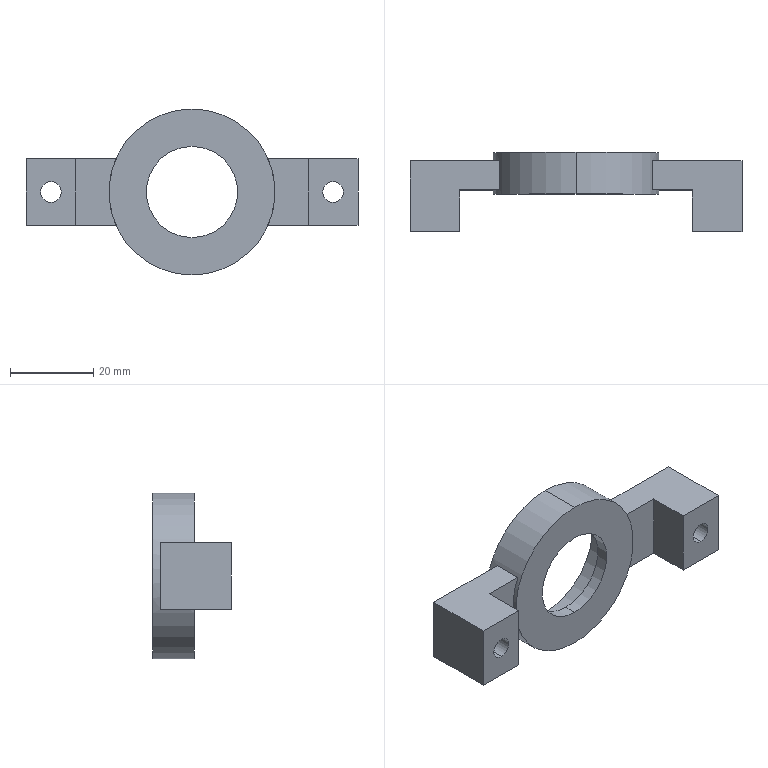Component | SolidWorks | BearingHousing-2 | 1 solid | 33 faces | box 80 x 19 x 40 mm | volume 12982 mm3 | plane 19 | cylinder 14 | commonest cylinder face diameters 10 x4 5 x4 32 x2 40 x2 22 x2 | material A-Glass Fiber
build123d program:
from build123d import *

# Parameters (mm, degrees)
BOSS_EXTRUDE1_DEPTH      = 7
BOSS_EXTRUDE1_DEPTH_BACK = 3
SKETCH1_R                = 20
SKETCH1_R_2              = 11
BOSS_EXTRUDE2_START      = -2
BOSS_EXTRUDE2_DEPTH      = 7
SKETCH3_W                = 12
SKETCH3_H                = 16
BOSS_EXTRUDE3_DEPTH      = 12
SKETCH4_R                = 2.5
CUT_EXTRUDE1_DEPTH       = 49.59
SKETCH5_R                = 5
CUT_EXTRUDE2_DEPTH       = 5
SKETCH6_R                = 16
CUT_EXTRUDE3_DEPTH       = 7


with BuildPart() as part:
    # Sketch1 → Boss-Extrude1 (new, two sides: drawn at the far end of the back side and taken through both)
    with BuildSketch(Plane(origin=(0, 0, 0), x_dir=(1, 0, 0), z_dir=(0, 1, 0)).offset(-BOSS_EXTRUDE1_DEPTH_BACK)):
        with Locations(Location((0, 0, 0), (0, 0, 270))):
            Circle(SKETCH1_R)
        with Locations(Location((0, 0, 0), (0, 0, 270))):
            Circle(SKETCH1_R_2, mode=Mode.SUBTRACT)
    extrude(amount=BOSS_EXTRUDE1_DEPTH + BOSS_EXTRUDE1_DEPTH_BACK)

    # Sketch2 → Boss-Extrude2 (add)
    with BuildSketch(Plane(origin=(0, 0, 0), x_dir=(1, 0, 0), z_dir=(0, 1, 0)).offset(BOSS_EXTRUDE2_START)):
        with BuildLine():
            Line((40, 8), (18.33, 8))
            ThreePointArc((18.33, 8), (20, 0), (18.33, -8))
            Line((18.33, -8), (40, -8))
            Line((40, -8), (40, 8))
        make_face()
    boss_extrude2 = extrude(amount=BOSS_EXTRUDE2_DEPTH)

    # Sketch3 → Boss-Extrude3 (add)
    with BuildSketch(Plane(origin=(0, 0, 0), x_dir=(1, 0, 0), z_dir=(0, 1, 0))):
        with Locations((34, 0)):
            Rectangle(SKETCH3_W, SKETCH3_H)
    boss_extrude3 = extrude(amount=-BOSS_EXTRUDE3_DEPTH)

    # Sketch4 → Cut-Extrude1 (cut, through all)
    with BuildSketch(Plane.XZ.offset(12)):
        with Locations(Location((34, 0, 0), (0, 0, 270))):
            Circle(SKETCH4_R)
    cut_extrude1 = extrude(amount=-CUT_EXTRUDE1_DEPTH, mode=Mode.SUBTRACT)

    # Sketch5 → Cut-Extrude2 (cut)
    with BuildSketch(Plane(origin=(0, 5, 0), x_dir=(1, 0, 0), z_dir=(0, 1, 0))):
        with Locations(Location((34, 0, 0), (0, 0, 270))):
            Circle(SKETCH5_R)
    cut_extrude2 = extrude(amount=-CUT_EXTRUDE2_DEPTH, mode=Mode.SUBTRACT)

    # Mirror1: Boss-Extrude2, Boss-Extrude3, Cut-Extrude1, Cut-Extrude2 across plane
    add(boss_extrude2.mirror(Plane(origin=(0, 0, 0), x_dir=(0, 0, 1), z_dir=(1, 0, 0))))
    add(boss_extrude3.mirror(Plane(origin=(0, 0, 0), x_dir=(0, 0, 1), z_dir=(1, 0, 0))))
    add(cut_extrude1.mirror(Plane(origin=(0, 0, 0), x_dir=(0, 0, 1), z_dir=(1, 0, 0))), mode=Mode.SUBTRACT)
    add(cut_extrude2.mirror(Plane(origin=(0, 0, 0), x_dir=(0, 0, 1), z_dir=(1, 0, 0))), mode=Mode.SUBTRACT)

    # Sketch6 → Cut-Extrude3 (cut)
    with BuildSketch(Plane(origin=(0, 7, 0), x_dir=(1, 0, 0), z_dir=(0, 1, 0))):
        with Locations(Location((0, 0, 0), (0, 0, 270))):
            Circle(SKETCH6_R)
    extrude(amount=-CUT_EXTRUDE3_DEPTH, mode=Mode.SUBTRACT)


solid = part.part

# Placed as in the assembly
solid = solid.moved(Location((-96.534, 130.266, -166.507), (0, 0, 0)))
STEP:
#1=COLOUR_RGB('',0.7922,0.8196,0.9333);
#2=FILL_AREA_STYLE_COLOUR('',#1);
#3=FILL_AREA_STYLE('',(#2));
#4=SURFACE_STYLE_FILL_AREA(#3);
#5=SURFACE_SIDE_STYLE('',(#4));
#6=SURFACE_STYLE_USAGE(.BOTH.,#5);
#7=PRESENTATION_STYLE_ASSIGNMENT((#6));
#8=CARTESIAN_POINT('',(-3.801,5.129,-7.185));
#9=VERTEX_POINT('',#8);
#10=CARTESIAN_POINT('',(-3.801,5.129,-5.925));
#11=VERTEX_POINT('',#10);
#12=CARTESIAN_POINT('',(-3.801,5.129,-6.555));
#13=DIRECTION('',(0.,1.,0.));
#14=DIRECTION('',(0.,0.,1.));
#15=AXIS2_PLACEMENT_3D('',#12,#13,#14);
#16=CIRCLE('',#15,0.6299);
#17=EDGE_CURVE('',#9,#11,#16,.T.);
#18=ORIENTED_EDGE('',*,*,#17,.F.);
#19=CARTESIAN_POINT('',(-3.801,5.404,-7.185));
#20=VERTEX_POINT('',#19);
#21=CARTESIAN_POINT('',(-3.801,5.129,-7.185));
#22=DIRECTION('',(0.,1.,0.));
#23=VECTOR('',#22,39.37);
#24=LINE('',#21,#23);
#25=EDGE_CURVE('',#9,#20,#24,.T.);
#26=ORIENTED_EDGE('',*,*,#25,.T.);
#27=CARTESIAN_POINT('',(-3.801,5.404,-5.925));
#28=VERTEX_POINT('',#27);
#29=CARTESIAN_POINT('',(-3.801,5.404,-6.555));
#30=DIRECTION('',(0.,1.,0.));
#31=DIRECTION('',(0.,0.,1.));
#32=AXIS2_PLACEMENT_3D('',#29,#30,#31);
#33=CIRCLE('',#32,0.6299);
#34=EDGE_CURVE('',#20,#28,#33,.T.);
#35=ORIENTED_EDGE('',*,*,#34,.T.);
#36=CARTESIAN_POINT('',(-3.801,5.129,-5.925));
#37=DIRECTION('',(0.,1.,0.));
#38=VECTOR('',#37,39.37);
#39=LINE('',#36,#38);
#40=EDGE_CURVE('',#11,#28,#39,.T.);
#41=ORIENTED_EDGE('',*,*,#40,.F.);
#42=EDGE_LOOP('',(#18,#26,#35,#41));
#43=FACE_OUTER_BOUND('',#42,.T.);
#44=CARTESIAN_POINT('',(-3.801,5.129,-6.555));
#45=DIRECTION('',(0.,1.,0.));
#46=DIRECTION('',(0.,0.,1.));
#47=AXIS2_PLACEMENT_3D('',#44,#45,#46);
#48=CYLINDRICAL_SURFACE('',#47,0.6299);
#49=ADVANCED_FACE('',(#43),#48,.F.);
#50=CARTESIAN_POINT('',(-5.139,5.129,-6.359));
#51=VERTEX_POINT('',#50);
#52=CARTESIAN_POINT('',(-5.139,5.129,-6.752));
#53=VERTEX_POINT('',#52);
#54=CARTESIAN_POINT('',(-5.139,5.129,-6.555));
#55=DIRECTION('',(0.,-1.,0.));
#56=DIRECTION('',(0.,0.,1.));
#57=AXIS2_PLACEMENT_3D('',#54,#55,#56);
#58=CIRCLE('',#57,0.1969);
#59=EDGE_CURVE('',#51,#53,#58,.T.);
#60=ORIENTED_EDGE('',*,*,#59,.T.);
#61=CARTESIAN_POINT('',(-5.139,5.325,-6.752));
#62=VERTEX_POINT('',#61);
#63=CARTESIAN_POINT('',(-5.139,5.129,-6.752));
#64=DIRECTION('',(0.,1.,0.));
#65=VECTOR('',#64,39.37);
#66=LINE('',#63,#65);
#67=EDGE_CURVE('',#53,#62,#66,.T.);
#68=ORIENTED_EDGE('',*,*,#67,.T.);
#69=CARTESIAN_POINT('',(-5.139,5.325,-6.359));
#70=VERTEX_POINT('',#69);
#71=CARTESIAN_POINT('',(-5.139,5.325,-6.555));
#72=DIRECTION('',(0.,-1.,0.));
#73=DIRECTION('',(0.,0.,1.));
#74=AXIS2_PLACEMENT_3D('',#71,#72,#73);
#75=CIRCLE('',#74,0.1969);
#76=EDGE_CURVE('',#70,#62,#75,.T.);
#77=ORIENTED_EDGE('',*,*,#76,.F.);
#78=CARTESIAN_POINT('',(-5.139,5.129,-6.359));
#79=DIRECTION('',(0.,1.,0.));
#80=VECTOR('',#79,39.37);
#81=LINE('',#78,#80);
#82=EDGE_CURVE('',#51,#70,#81,.T.);
#83=ORIENTED_EDGE('',*,*,#82,.F.);
#84=EDGE_LOOP('',(#60,#68,#77,#83));
#85=FACE_OUTER_BOUND('',#84,.T.);
#86=CARTESIAN_POINT('',(-5.139,5.129,-6.555));
#87=DIRECTION('',(0.,1.,0.));
#88=DIRECTION('',(0.,0.,1.));
#89=AXIS2_PLACEMENT_3D('',#86,#87,#88);
#90=CYLINDRICAL_SURFACE('',#89,0.1969);
#91=ADVANCED_FACE('',(#85),#90,.F.);
#92=CARTESIAN_POINT('',(-2.462,5.129,-6.752));
#93=VERTEX_POINT('',#92);
#94=CARTESIAN_POINT('',(-2.462,5.129,-6.359));
#95=VERTEX_POINT('',#94);
#96=CARTESIAN_POINT('',(-2.462,5.129,-6.555));
#97=DIRECTION('',(0.,1.,0.));
#98=DIRECTION('',(0.,0.,1.));
#99=AXIS2_PLACEMENT_3D('',#96,#97,#98);
#100=CIRCLE('',#99,0.1969);
#101=EDGE_CURVE('',#93,#95,#100,.T.);
#102=ORIENTED_EDGE('',*,*,#101,.F.);
#103=CARTESIAN_POINT('',(-2.462,5.325,-6.752));
#104=VERTEX_POINT('',#103);
#105=CARTESIAN_POINT('',(-2.462,5.129,-6.752));
#106=DIRECTION('',(0.,1.,0.));
#107=VECTOR('',#106,39.37);
#108=LINE('',#105,#107);
#109=EDGE_CURVE('',#93,#104,#108,.T.);
#110=ORIENTED_EDGE('',*,*,#109,.T.);
#111=CARTESIAN_POINT('',(-2.462,5.325,-6.359));
#112=VERTEX_POINT('',#111);
#113=CARTESIAN_POINT('',(-2.462,5.325,-6.555));
#114=DIRECTION('',(0.,1.,0.));
#115=DIRECTION('',(0.,0.,1.));
#116=AXIS2_PLACEMENT_3D('',#113,#114,#115);
#117=CIRCLE('',#116,0.1969);
#118=EDGE_CURVE('',#104,#112,#117,.T.);
#119=ORIENTED_EDGE('',*,*,#118,.T.);
#120=CARTESIAN_POINT('',(-2.462,5.129,-6.359));
#121=DIRECTION('',(0.,1.,0.));
#122=VECTOR('',#121,39.37);
#123=LINE('',#120,#122);
#124=EDGE_CURVE('',#95,#112,#123,.T.);
#125=ORIENTED_EDGE('',*,*,#124,.F.);
#126=EDGE_LOOP('',(#102,#110,#119,#125));
#127=FACE_OUTER_BOUND('',#126,.T.);
#128=CARTESIAN_POINT('',(-2.462,5.129,-6.555));
#129=DIRECTION('',(0.,1.,0.));
#130=DIRECTION('',(0.,0.,1.));
#131=AXIS2_PLACEMENT_3D('',#128,#129,#130);
#132=CYLINDRICAL_SURFACE('',#131,0.1969);
#133=ADVANCED_FACE('',(#127),#132,.F.);
#134=CARTESIAN_POINT('',(-3.079,5.325,-6.87));
#135=VERTEX_POINT('',#134);
#136=CARTESIAN_POINT('',(-3.079,5.325,-6.24));
#137=VERTEX_POINT('',#136);
#138=CARTESIAN_POINT('',(-3.801,5.325,-6.555));
#139=DIRECTION('',(0.,-1.,0.));
#140=DIRECTION('',(0.,0.,1.));
#141=AXIS2_PLACEMENT_3D('',#138,#139,#140);
#142=CIRCLE('',#141,0.7874);
#143=EDGE_CURVE('',#135,#137,#142,.T.);
#144=ORIENTED_EDGE('',*,*,#143,.F.);
#145=CARTESIAN_POINT('',(-3.079,5.05,-6.87));
#146=VERTEX_POINT('',#145);
#147=CARTESIAN_POINT('',(-3.079,5.325,-6.87));
#148=DIRECTION('',(0.,-1.,0.));
#149=VECTOR('',#148,39.37);
#150=LINE('',#147,#149);
#151=EDGE_CURVE('',#135,#146,#150,.T.);
#152=ORIENTED_EDGE('',*,*,#151,.T.);
#153=CARTESIAN_POINT('',(-3.079,5.05,-6.24));
#154=VERTEX_POINT('',#153);
#155=CARTESIAN_POINT('',(-3.801,5.05,-6.555));
#156=DIRECTION('',(0.,-1.,0.));
#157=DIRECTION('',(0.,0.,1.));
#158=AXIS2_PLACEMENT_3D('',#155,#156,#157);
#159=CIRCLE('',#158,0.7874);
#160=EDGE_CURVE('',#146,#154,#159,.T.);
#161=ORIENTED_EDGE('',*,*,#160,.T.);
#162=CARTESIAN_POINT('',(-3.079,5.325,-6.24));
#163=DIRECTION('',(0.,-1.,0.));
#164=VECTOR('',#163,39.37);
#165=LINE('',#162,#164);
#166=EDGE_CURVE('',#137,#154,#165,.T.);
#167=ORIENTED_EDGE('',*,*,#166,.F.);
#168=EDGE_LOOP('',(#144,#152,#161,#167));
#169=FACE_BOUND('',#168,.T.);
#170=CARTESIAN_POINT('',(-3.801,5.01,-5.768));
#171=VERTEX_POINT('',#170);
#172=CARTESIAN_POINT('',(-3.801,5.01,-7.343));
#173=VERTEX_POINT('',#172);
#174=CARTESIAN_POINT('',(-3.801,5.01,-6.555));
#175=DIRECTION('',(0.,1.,0.));
#176=DIRECTION('',(0.,0.,1.));
#177=AXIS2_PLACEMENT_3D('',#174,#175,#176);
#178=CIRCLE('',#177,0.7874);
#179=EDGE_CURVE('',#171,#173,#178,.T.);
#180=ORIENTED_EDGE('',*,*,#179,.T.);
#181=CARTESIAN_POINT('',(-3.801,5.404,-7.343));
#182=VERTEX_POINT('',#181);
#183=CARTESIAN_POINT('',(-3.801,5.01,-7.343));
#184=DIRECTION('',(0.,1.,0.));
#185=VECTOR('',#184,39.37);
#186=LINE('',#183,#185);
#187=EDGE_CURVE('',#173,#182,#186,.T.);
#188=ORIENTED_EDGE('',*,*,#187,.T.);
#189=CARTESIAN_POINT('',(-3.801,5.404,-5.768));
#190=VERTEX_POINT('',#189);
#191=CARTESIAN_POINT('',(-3.801,5.404,-6.555));
#192=DIRECTION('',(0.,1.,0.));
#193=DIRECTION('',(0.,0.,1.));
#194=AXIS2_PLACEMENT_3D('',#191,#192,#193);
#195=CIRCLE('',#194,0.7874);
#196=EDGE_CURVE('',#190,#182,#195,.T.);
#197=ORIENTED_EDGE('',*,*,#196,.F.);
#198=CARTESIAN_POINT('',(-3.801,5.01,-5.768));
#199=DIRECTION('',(0.,1.,0.));
#200=VECTOR('',#199,39.37);
#201=LINE('',#198,#200);
#202=EDGE_CURVE('',#171,#190,#201,.T.);
#203=ORIENTED_EDGE('',*,*,#202,.F.);
#204=EDGE_LOOP('',(#180,#188,#197,#203));
#205=FACE_OUTER_BOUND('',#204,.T.);
#206=CARTESIAN_POINT('',(-3.801,5.01,-6.555));
#207=DIRECTION('',(0.,1.,0.));
#208=DIRECTION('',(0.,0.,1.));
#209=AXIS2_PLACEMENT_3D('',#206,#207,#208);
#210=CYLINDRICAL_SURFACE('',#209,0.7874);
#211=ADVANCED_FACE('',(#169,#205),#210,.T.);
#212=CARTESIAN_POINT('',(-2.462,5.129,-6.457));
#213=VERTEX_POINT('',#212);
#214=CARTESIAN_POINT('',(-2.462,5.129,-6.654));
#215=VERTEX_POINT('',#214);
#216=CARTESIAN_POINT('',(-2.462,5.129,-6.555));
#217=DIRECTION('',(0.,-1.,0.));
#218=DIRECTION('',(0.,0.,1.));
#219=AXIS2_PLACEMENT_3D('',#216,#217,#218);
#220=CIRCLE('',#219,0.09843);
#221=EDGE_CURVE('',#213,#215,#220,.T.);
#222=ORIENTED_EDGE('',*,*,#221,.F.);
#223=CARTESIAN_POINT('',(-2.462,4.656,-6.457));
#224=VERTEX_POINT('',#223);
#225=CARTESIAN_POINT('',(-2.462,5.404,-6.457));
#226=DIRECTION('',(0.,-1.,0.));
#227=VECTOR('',#226,39.37);
#228=LINE('',#225,#227);
#229=EDGE_CURVE('',#213,#224,#228,.T.);
#230=ORIENTED_EDGE('',*,*,#229,.T.);
#231=CARTESIAN_POINT('',(-2.462,4.656,-6.654));
#232=VERTEX_POINT('',#231);
#233=CARTESIAN_POINT('',(-2.462,4.656,-6.555));
#234=DIRECTION('',(0.,-1.,0.));
#235=DIRECTION('',(0.,0.,-1.));
#236=AXIS2_PLACEMENT_3D('',#233,#234,#235);
#237=CIRCLE('',#236,0.09843);
#238=EDGE_CURVE('',#224,#232,#237,.T.);
#239=ORIENTED_EDGE('',*,*,#238,.T.);
#240=CARTESIAN_POINT('',(-2.462,5.404,-6.654));
#241=DIRECTION('',(0.,-1.,0.));
#242=VECTOR('',#241,39.37);
#243=LINE('',#240,#242);
#244=EDGE_CURVE('',#215,#232,#243,.T.);
#245=ORIENTED_EDGE('',*,*,#244,.F.);
#246=EDGE_LOOP('',(#222,#230,#239,#245));
#247=FACE_OUTER_BOUND('',#246,.T.);
#248=CARTESIAN_POINT('',(-2.462,5.404,-6.555));
#249=DIRECTION('',(0.,-1.,0.));
#250=DIRECTION('',(0.,0.,-1.));
#251=AXIS2_PLACEMENT_3D('',#248,#249,#250);
#252=CYLINDRICAL_SURFACE('',#251,0.09843);
#253=ADVANCED_FACE('',(#247),#252,.F.);
#254=CARTESIAN_POINT('',(-5.139,5.129,-6.654));
#255=VERTEX_POINT('',#254);
#256=CARTESIAN_POINT('',(-5.139,5.129,-6.457));
#257=VERTEX_POINT('',#256);
#258=CARTESIAN_POINT('',(-5.139,5.129,-6.555));
#259=DIRECTION('',(0.,1.,0.));
#260=DIRECTION('',(0.,0.,1.));
#261=AXIS2_PLACEMENT_3D('',#258,#259,#260);
#262=CIRCLE('',#261,0.09843);
#263=EDGE_CURVE('',#255,#257,#262,.T.);
#264=ORIENTED_EDGE('',*,*,#263,.T.);
#265=CARTESIAN_POINT('',(-5.139,4.656,-6.457));
#266=VERTEX_POINT('',#265);
#267=CARTESIAN_POINT('',(-5.139,5.404,-6.457));
#268=DIRECTION('',(0.,-1.,0.));
#269=VECTOR('',#268,39.37);
#270=LINE('',#267,#269);
#271=EDGE_CURVE('',#257,#266,#270,.T.);
#272=ORIENTED_EDGE('',*,*,#271,.T.);
#273=CARTESIAN_POINT('',(-5.139,4.656,-6.654));
#274=VERTEX_POINT('',#273);
#275=CARTESIAN_POINT('',(-5.139,4.656,-6.555));
#276=DIRECTION('',(0.,1.,0.));
#277=DIRECTION('',(0.,0.,-1.));
#278=AXIS2_PLACEMENT_3D('',#275,#276,#277);
#279=CIRCLE('',#278,0.09843);
#280=EDGE_CURVE('',#274,#266,#279,.T.);
#281=ORIENTED_EDGE('',*,*,#280,.F.);
#282=CARTESIAN_POINT('',(-5.139,5.404,-6.654));
#283=DIRECTION('',(0.,-1.,0.));
#284=VECTOR('',#283,39.37);
#285=LINE('',#282,#284);
#286=EDGE_CURVE('',#255,#274,#285,.T.);
#287=ORIENTED_EDGE('',*,*,#286,.F.);
#288=EDGE_LOOP('',(#264,#272,#281,#287));
#289=FACE_OUTER_BOUND('',#288,.T.);
#290=CARTESIAN_POINT('',(-5.139,5.404,-6.555));
#291=DIRECTION('',(0.,-1.,0.));
#292=DIRECTION('',(0.,0.,-1.));
#293=AXIS2_PLACEMENT_3D('',#290,#291,#292);
#294=CYLINDRICAL_SURFACE('',#293,0.09843);
#295=ADVANCED_FACE('',(#289),#294,.F.);
#296=CARTESIAN_POINT('',(-3.801,5.01,-6.988));
#297=VERTEX_POINT('',#296);
#298=CARTESIAN_POINT('',(-3.801,5.01,-6.122));
#299=VERTEX_POINT('',#298);
#300=CARTESIAN_POINT('',(-3.801,5.01,-6.555));
#301=DIRECTION('',(0.,1.,0.));
#302=DIRECTION('',(0.,0.,1.));
#303=AXIS2_PLACEMENT_3D('',#300,#301,#302);
#304=CIRCLE('',#303,0.4331);
#305=EDGE_CURVE('',#297,#299,#304,.T.);
#306=ORIENTED_EDGE('',*,*,#305,.F.);
#307=CARTESIAN_POINT('',(-3.801,5.129,-6.988));
#308=VERTEX_POINT('',#307);
#309=CARTESIAN_POINT('',(-3.801,5.01,-6.988));
#310=DIRECTION('',(0.,1.,0.));
#311=VECTOR('',#310,39.37);
#312=LINE('',#309,#311);
#313=EDGE_CURVE('',#297,#308,#312,.T.);
#314=ORIENTED_EDGE('',*,*,#313,.T.);
#315=CARTESIAN_POINT('',(-3.801,5.129,-6.122));
#316=VERTEX_POINT('',#315);
#317=CARTESIAN_POINT('',(-3.801,5.129,-6.555));
#318=DIRECTION('',(0.,-1.,0.));
#319=DIRECTION('',(0.,0.,1.));
#320=AXIS2_PLACEMENT_3D('',#317,#318,#319);
#321=CIRCLE('',#320,0.4331);
#322=EDGE_CURVE('',#316,#308,#321,.T.);
#323=ORIENTED_EDGE('',*,*,#322,.F.);
#324=CARTESIAN_POINT('',(-3.801,5.01,-6.122));
#325=DIRECTION('',(0.,1.,0.));
#326=VECTOR('',#325,39.37);
#327=LINE('',#324,#326);
#328=EDGE_CURVE('',#299,#316,#327,.T.);
#329=ORIENTED_EDGE('',*,*,#328,.F.);
#330=EDGE_LOOP('',(#306,#314,#323,#329));
#331=FACE_OUTER_BOUND('',#330,.T.);
#332=CARTESIAN_POINT('',(-3.801,5.01,-6.555));
#333=DIRECTION('',(0.,1.,0.));
#334=DIRECTION('',(0.,0.,1.));
#335=AXIS2_PLACEMENT_3D('',#332,#333,#334);
#336=CYLINDRICAL_SURFACE('',#335,0.4331);
#337=ADVANCED_FACE('',(#331),#336,.F.);
#338=ORIENTED_EDGE('',*,*,#313,.F.);
#339=CARTESIAN_POINT('',(-3.801,5.01,-6.555));
#340=DIRECTION('',(0.,1.,0.));
#341=DIRECTION('',(0.,0.,1.));
#342=AXIS2_PLACEMENT_3D('',#339,#340,#341);
#343=CIRCLE('',#342,0.4331);
#344=EDGE_CURVE('',#299,#297,#343,.T.);
#345=ORIENTED_EDGE('',*,*,#344,.F.);
#346=ORIENTED_EDGE('',*,*,#328,.T.);
#347=CARTESIAN_POINT('',(-3.801,5.129,-6.555));
#348=DIRECTION('',(0.,-1.,0.));
#349=DIRECTION('',(0.,0.,1.));
#350=AXIS2_PLACEMENT_3D('',#347,#348,#349);
#351=CIRCLE('',#350,0.4331);
#352=EDGE_CURVE('',#308,#316,#351,.T.);
#353=ORIENTED_EDGE('',*,*,#352,.F.);
#354=EDGE_LOOP('',(#338,#345,#346,#353));
#355=FACE_OUTER_BOUND('',#354,.T.);
#356=CARTESIAN_POINT('',(-3.801,5.01,-6.555));
#357=DIRECTION('',(0.,1.,0.));
#358=DIRECTION('',(0.,0.,1.));
#359=AXIS2_PLACEMENT_3D('',#356,#357,#358);
#360=CYLINDRICAL_SURFACE('',#359,0.4331);
#361=ADVANCED_FACE('',(#355),#360,.F.);
#362=CARTESIAN_POINT('',(-4.522,5.325,-6.87));
#363=VERTEX_POINT('',#362);
#364=CARTESIAN_POINT('',(-4.522,5.325,-6.24));
#365=VERTEX_POINT('',#364);
#366=CARTESIAN_POINT('',(-3.801,5.325,-6.555));
#367=DIRECTION('',(0.,1.,0.));
#368=DIRECTION('',(0.,0.,1.));
#369=AXIS2_PLACEMENT_3D('',#366,#367,#368);
#370=CIRCLE('',#369,0.7874);
#371=EDGE_CURVE('',#363,#365,#370,.T.);
#372=ORIENTED_EDGE('',*,*,#371,.F.);
#373=CARTESIAN_POINT('',(-5.375,5.325,-6.87));
#374=VERTEX_POINT('',#373);
#375=CARTESIAN_POINT('',(-5.375,5.325,-6.87));
#376=DIRECTION('',(1.,0.,0.));
#377=VECTOR('',#376,39.37);
#378=LINE('',#375,#377);
#379=EDGE_CURVE('',#374,#363,#378,.T.);
#380=ORIENTED_EDGE('',*,*,#379,.F.);
#381=CARTESIAN_POINT('',(-5.375,5.325,-6.24));
#382=VERTEX_POINT('',#381);
#383=CARTESIAN_POINT('',(-5.375,5.325,-6.87));
#384=DIRECTION('',(0.,0.,-1.));
#385=VECTOR('',#384,39.37);
#386=LINE('',#383,#385);
#387=EDGE_CURVE('',#382,#374,#386,.T.);
#388=ORIENTED_EDGE('',*,*,#387,.F.);
#389=CARTESIAN_POINT('',(-5.375,5.325,-6.24));
#390=DIRECTION('',(-1.,0.,0.));
#391=VECTOR('',#390,39.37);
#392=LINE('',#389,#391);
#393=EDGE_CURVE('',#365,#382,#392,.T.);
#394=ORIENTED_EDGE('',*,*,#393,.F.);
#395=EDGE_LOOP('',(#372,#380,#388,#394));
#396=FACE_OUTER_BOUND('',#395,.T.);
#397=ORIENTED_EDGE('',*,*,#76,.T.);
#398=CARTESIAN_POINT('',(-5.139,5.325,-6.555));
#399=DIRECTION('',(0.,-1.,0.));
#400=DIRECTION('',(0.,0.,1.));
#401=AXIS2_PLACEMENT_3D('',#398,#399,#400);
#402=CIRCLE('',#401,0.1969);
#403=EDGE_CURVE('',#62,#70,#402,.T.);
#404=ORIENTED_EDGE('',*,*,#403,.T.);
#405=EDGE_LOOP('',(#397,#404));
#406=FACE_BOUND('',#405,.T.);
#407=CARTESIAN_POINT('',(-3.801,5.325,-6.555));
#408=DIRECTION('',(0.,1.,0.));
#409=DIRECTION('',(0.,0.,1.));
#410=AXIS2_PLACEMENT_3D('',#407,#408,#409);
#411=PLANE('',#410);
#412=ADVANCED_FACE('',(#396,#406),#411,.T.);
#413=ORIENTED_EDGE('',*,*,#271,.F.);
#414=CARTESIAN_POINT('',(-5.139,5.129,-6.555));
#415=DIRECTION('',(0.,1.,0.));
#416=DIRECTION('',(0.,0.,1.));
#417=AXIS2_PLACEMENT_3D('',#414,#415,#416);
#418=CIRCLE('',#417,0.09843);
#419=EDGE_CURVE('',#257,#255,#418,.T.);
#420=ORIENTED_EDGE('',*,*,#419,.T.);
#421=ORIENTED_EDGE('',*,*,#286,.T.);
#422=CARTESIAN_POINT('',(-5.139,4.656,-6.555));
#423=DIRECTION('',(0.,1.,0.));
#424=DIRECTION('',(0.,0.,-1.));
#425=AXIS2_PLACEMENT_3D('',#422,#423,#424);
#426=CIRCLE('',#425,0.09843);
#427=EDGE_CURVE('',#266,#274,#426,.T.);
#428=ORIENTED_EDGE('',*,*,#427,.F.);
#429=EDGE_LOOP('',(#413,#420,#421,#428));
#430=FACE_OUTER_BOUND('',#429,.T.);
#431=CARTESIAN_POINT('',(-5.139,5.404,-6.555));
#432=DIRECTION('',(0.,-1.,0.));
#433=DIRECTION('',(0.,0.,-1.));
#434=AXIS2_PLACEMENT_3D('',#431,#432,#433);
#435=CYLINDRICAL_SURFACE('',#434,0.09843);
#436=ADVANCED_FACE('',(#430),#435,.F.);
#437=CARTESIAN_POINT('',(-5.375,4.656,-6.24));
#438=VERTEX_POINT('',#437);
#439=CARTESIAN_POINT('',(-5.375,4.656,-6.87));
#440=VERTEX_POINT('',#439);
#441=CARTESIAN_POINT('',(-5.375,4.656,-6.87));
#442=DIRECTION('',(0.,0.,-1.));
#443=VECTOR('',#442,39.37);
#444=LINE('',#441,#443);
#445=EDGE_CURVE('',#438,#440,#444,.T.);
#446=ORIENTED_EDGE('',*,*,#445,.T.);
#447=CARTESIAN_POINT('',(-4.903,4.656,-6.87));
#448=VERTEX_POINT('',#447);
#449=CARTESIAN_POINT('',(-5.375,4.656,-6.87));
#450=DIRECTION('',(1.,0.,0.));
#451=VECTOR('',#450,39.37);
#452=LINE('',#449,#451);
#453=EDGE_CURVE('',#440,#448,#452,.T.);
#454=ORIENTED_EDGE('',*,*,#453,.T.);
#455=CARTESIAN_POINT('',(-4.903,4.656,-6.24));
#456=VERTEX_POINT('',#455);
#457=CARTESIAN_POINT('',(-4.903,4.656,-6.87));
#458=DIRECTION('',(0.,0.,1.));
#459=VECTOR('',#458,39.37);
#460=LINE('',#457,#459);
#461=EDGE_CURVE('',#448,#456,#460,.T.);
#462=ORIENTED_EDGE('',*,*,#461,.T.);
#463=CARTESIAN_POINT('',(-5.375,4.656,-6.24));
#464=DIRECTION('',(-1.,0.,0.));
#465=VECTOR('',#464,39.37);
#466=LINE('',#463,#465);
#467=EDGE_CURVE('',#456,#438,#466,.T.);
#468=ORIENTED_EDGE('',*,*,#467,.T.);
#469=EDGE_LOOP('',(#446,#454,#462,#468));
#470=FACE_OUTER_BOUND('',#469,.T.);
#471=ORIENTED_EDGE('',*,*,#280,.T.);
#472=ORIENTED_EDGE('',*,*,#427,.T.);
#473=EDGE_LOOP('',(#471,#472));
#474=FACE_BOUND('',#473,.T.);
#475=CARTESIAN_POINT('',(-3.801,4.656,-6.555));
#476=DIRECTION('',(0.,-1.,0.));
#477=DIRECTION('',(0.,0.,-1.));
#478=AXIS2_PLACEMENT_3D('',#475,#476,#477);
#479=PLANE('',#478);
#480=ADVANCED_FACE('',(#470,#474),#479,.T.);
#481=CARTESIAN_POINT('',(-4.903,5.05,-6.87));
#482=VERTEX_POINT('',#481);
#483=CARTESIAN_POINT('',(-4.903,5.05,-6.24));
#484=VERTEX_POINT('',#483);
#485=CARTESIAN_POINT('',(-4.903,5.05,-6.555));
#486=DIRECTION('',(0.,0.,1.));
#487=VECTOR('',#486,39.37);
#488=LINE('',#485,#487);
#489=EDGE_CURVE('',#482,#484,#488,.T.);
#490=ORIENTED_EDGE('',*,*,#489,.F.);
#491=CARTESIAN_POINT('',(-4.522,5.05,-6.87));
#492=VERTEX_POINT('',#491);
#493=CARTESIAN_POINT('',(-5.375,5.05,-6.87));
#494=DIRECTION('',(1.,0.,0.));
#495=VECTOR('',#494,39.37);
#496=LINE('',#493,#495);
#497=EDGE_CURVE('',#482,#492,#496,.T.);
#498=ORIENTED_EDGE('',*,*,#497,.T.);
#499=CARTESIAN_POINT('',(-4.522,5.05,-6.24));
#500=VERTEX_POINT('',#499);
#501=CARTESIAN_POINT('',(-3.801,5.05,-6.555));
#502=DIRECTION('',(0.,1.,0.));
#503=DIRECTION('',(0.,0.,1.));
#504=AXIS2_PLACEMENT_3D('',#501,#502,#503);
#505=CIRCLE('',#504,0.7874);
#506=EDGE_CURVE('',#492,#500,#505,.T.);
#507=ORIENTED_EDGE('',*,*,#506,.T.);
#508=CARTESIAN_POINT('',(-5.375,5.05,-6.24));
#509=DIRECTION('',(-1.,0.,0.));
#510=VECTOR('',#509,39.37);
#511=LINE('',#508,#510);
#512=EDGE_CURVE('',#500,#484,#511,.T.);
#513=ORIENTED_EDGE('',*,*,#512,.T.);
#514=EDGE_LOOP('',(#490,#498,#507,#513));
#515=FACE_OUTER_BOUND('',#514,.T.);
#516=CARTESIAN_POINT('',(-3.801,5.05,-6.555));
#517=DIRECTION('',(0.,1.,0.));
#518=DIRECTION('',(0.,0.,1.));
#519=AXIS2_PLACEMENT_3D('',#516,#517,#518);
#520=PLANE('',#519);
#521=ADVANCED_FACE('',(#515),#520,.F.);
#522=ORIENTED_EDGE('',*,*,#229,.F.);
#523=CARTESIAN_POINT('',(-2.462,5.129,-6.555));
#524=DIRECTION('',(0.,-1.,0.));
#525=DIRECTION('',(0.,0.,1.));
#526=AXIS2_PLACEMENT_3D('',#523,#524,#525);
#527=CIRCLE('',#526,0.09843);
#528=EDGE_CURVE('',#215,#213,#527,.T.);
#529=ORIENTED_EDGE('',*,*,#528,.F.);
#530=ORIENTED_EDGE('',*,*,#244,.T.);
#531=CARTESIAN_POINT('',(-2.462,4.656,-6.555));
#532=DIRECTION('',(0.,-1.,0.));
#533=DIRECTION('',(0.,0.,-1.));
#534=AXIS2_PLACEMENT_3D('',#531,#532,#533);
#535=CIRCLE('',#534,0.09843);
#536=EDGE_CURVE('',#232,#224,#535,.T.);
#537=ORIENTED_EDGE('',*,*,#536,.T.);
#538=EDGE_LOOP('',(#522,#529,#530,#537));
#539=FACE_OUTER_BOUND('',#538,.T.);
#540=CARTESIAN_POINT('',(-2.462,5.404,-6.555));
#541=DIRECTION('',(0.,-1.,0.));
#542=DIRECTION('',(0.,0.,-1.));
#543=AXIS2_PLACEMENT_3D('',#540,#541,#542);
#544=CYLINDRICAL_SURFACE('',#543,0.09843);
#545=ADVANCED_FACE('',(#539),#544,.F.);
#546=ORIENTED_EDGE('',*,*,#187,.F.);
#547=CARTESIAN_POINT('',(-3.801,5.01,-6.555));
#548=DIRECTION('',(0.,1.,0.));
#549=DIRECTION('',(0.,0.,1.));
#550=AXIS2_PLACEMENT_3D('',#547,#548,#549);
#551=CIRCLE('',#550,0.7874);
#552=EDGE_CURVE('',#173,#171,#551,.T.);
#553=ORIENTED_EDGE('',*,*,#552,.T.);
#554=ORIENTED_EDGE('',*,*,#202,.T.);
#555=CARTESIAN_POINT('',(-3.801,5.404,-6.555));
#556=DIRECTION('',(0.,1.,0.));
#557=DIRECTION('',(0.,0.,1.));
#558=AXIS2_PLACEMENT_3D('',#555,#556,#557);
#559=CIRCLE('',#558,0.7874);
#560=EDGE_CURVE('',#182,#190,#559,.T.);
#561=ORIENTED_EDGE('',*,*,#560,.F.);
#562=EDGE_LOOP('',(#546,#553,#554,#561));
#563=FACE_OUTER_BOUND('',#562,.T.);
#564=ORIENTED_EDGE('',*,*,#371,.T.);
#565=CARTESIAN_POINT('',(-4.522,5.325,-6.24));
#566=DIRECTION('',(0.,-1.,0.));
#567=VECTOR('',#566,39.37);
#568=LINE('',#565,#567);
#569=EDGE_CURVE('',#365,#500,#568,.T.);
#570=ORIENTED_EDGE('',*,*,#569,.T.);
#571=ORIENTED_EDGE('',*,*,#506,.F.);
#572=CARTESIAN_POINT('',(-4.522,5.325,-6.87));
#573=DIRECTION('',(0.,-1.,0.));
#574=VECTOR('',#573,39.37);
#575=LINE('',#572,#574);
#576=EDGE_CURVE('',#363,#492,#575,.T.);
#577=ORIENTED_EDGE('',*,*,#576,.F.);
#578=EDGE_LOOP('',(#564,#570,#571,#577));
#579=FACE_BOUND('',#578,.T.);
#580=CARTESIAN_POINT('',(-3.801,5.01,-6.555));
#581=DIRECTION('',(0.,1.,0.));
#582=DIRECTION('',(0.,0.,1.));
#583=AXIS2_PLACEMENT_3D('',#580,#581,#582);
#584=CYLINDRICAL_SURFACE('',#583,0.7874);
#585=ADVANCED_FACE('',(#563,#579),#584,.T.);
#586=ORIENTED_EDGE('',*,*,#344,.T.);
#587=ORIENTED_EDGE('',*,*,#305,.T.);
#588=EDGE_LOOP('',(#586,#587));
#589=FACE_BOUND('',#588,.T.);
#590=ORIENTED_EDGE('',*,*,#179,.F.);
#591=ORIENTED_EDGE('',*,*,#552,.F.);
#592=EDGE_LOOP('',(#590,#591));
#593=FACE_OUTER_BOUND('',#592,.T.);
#594=CARTESIAN_POINT('',(-3.801,5.01,-6.555));
#595=DIRECTION('',(0.,1.,0.));
#596=DIRECTION('',(0.,0.,1.));
#597=AXIS2_PLACEMENT_3D('',#594,#595,#596);
#598=PLANE('',#597);
#599=ADVANCED_FACE('',(#589,#593),#598,.F.);
#600=CARTESIAN_POINT('',(-3.801,5.404,-6.555));
#601=DIRECTION('',(0.,1.,0.));
#602=DIRECTION('',(0.,0.,1.));
#603=AXIS2_PLACEMENT_3D('',#600,#601,#602);
#604=CIRCLE('',#603,0.6299);
#605=EDGE_CURVE('',#28,#20,#604,.T.);
#606=ORIENTED_EDGE('',*,*,#605,.F.);
#607=ORIENTED_EDGE('',*,*,#34,.F.);
#608=EDGE_LOOP('',(#606,#607));
#609=FACE_BOUND('',#608,.T.);
#610=ORIENTED_EDGE('',*,*,#196,.T.);
#611=ORIENTED_EDGE('',*,*,#560,.T.);
#612=EDGE_LOOP('',(#610,#611));
#613=FACE_OUTER_BOUND('',#612,.T.);
#614=CARTESIAN_POINT('',(-3.801,5.404,-6.555));
#615=DIRECTION('',(0.,1.,0.));
#616=DIRECTION('',(0.,0.,1.));
#617=AXIS2_PLACEMENT_3D('',#614,#615,#616);
#618=PLANE('',#617);
#619=ADVANCED_FACE('',(#609,#613),#618,.T.);
#620=CARTESIAN_POINT('',(-2.698,5.05,-6.24));
#621=VERTEX_POINT('',#620);
#622=CARTESIAN_POINT('',(-2.226,5.05,-6.24));
#623=DIRECTION('',(1.,0.,0.));
#624=VECTOR('',#623,39.37);
#625=LINE('',#622,#624);
#626=EDGE_CURVE('',#154,#621,#625,.T.);
#627=ORIENTED_EDGE('',*,*,#626,.T.);
#628=CARTESIAN_POINT('',(-2.698,4.656,-6.24));
#629=VERTEX_POINT('',#628);
#630=CARTESIAN_POINT('',(-2.698,4.656,-6.24));
#631=DIRECTION('',(0.,1.,0.));
#632=VECTOR('',#631,39.37);
#633=LINE('',#630,#632);
#634=EDGE_CURVE('',#629,#621,#633,.T.);
#635=ORIENTED_EDGE('',*,*,#634,.F.);
#636=CARTESIAN_POINT('',(-2.226,4.656,-6.24));
#637=VERTEX_POINT('',#636);
#638=CARTESIAN_POINT('',(-2.226,4.656,-6.24));
#639=DIRECTION('',(1.,0.,0.));
#640=VECTOR('',#639,39.37);
#641=LINE('',#638,#640);
#642=EDGE_CURVE('',#629,#637,#641,.T.);
#643=ORIENTED_EDGE('',*,*,#642,.T.);
#644=CARTESIAN_POINT('',(-2.226,5.325,-6.24));
#645=VERTEX_POINT('',#644);
#646=CARTESIAN_POINT('',(-2.226,5.325,-6.24));
#647=DIRECTION('',(0.,-1.,0.));
#648=VECTOR('',#647,39.37);
#649=LINE('',#646,#648);
#650=EDGE_CURVE('',#645,#637,#649,.T.);
#651=ORIENTED_EDGE('',*,*,#650,.F.);
#652=CARTESIAN_POINT('',(-2.226,5.325,-6.24));
#653=DIRECTION('',(1.,0.,0.));
#654=VECTOR('',#653,39.37);
#655=LINE('',#652,#654);
#656=EDGE_CURVE('',#137,#645,#655,.T.);
#657=ORIENTED_EDGE('',*,*,#656,.F.);
#658=ORIENTED_EDGE('',*,*,#166,.T.);
#659=EDGE_LOOP('',(#627,#635,#643,#651,#657,#658));
#660=FACE_OUTER_BOUND('',#659,.T.);
#661=CARTESIAN_POINT('',(-2.226,5.325,-6.24));
#662=DIRECTION('',(0.,0.,-1.));
#663=DIRECTION('',(-1.,0.,-0.));
#664=AXIS2_PLACEMENT_3D('',#661,#662,#663);
#665=PLANE('',#664);
#666=ADVANCED_FACE('',(#660),#665,.F.);
#667=CARTESIAN_POINT('',(-2.226,4.656,-6.87));
#668=VERTEX_POINT('',#667);
#669=CARTESIAN_POINT('',(-2.226,4.656,-6.87));
#670=DIRECTION('',(0.,0.,-1.));
#671=VECTOR('',#670,39.37);
#672=LINE('',#669,#671);
#673=EDGE_CURVE('',#637,#668,#672,.T.);
#674=ORIENTED_EDGE('',*,*,#673,.T.);
#675=CARTESIAN_POINT('',(-2.226,5.325,-6.87));
#676=VERTEX_POINT('',#675);
#677=CARTESIAN_POINT('',(-2.226,5.325,-6.87));
#678=DIRECTION('',(0.,-1.,0.));
#679=VECTOR('',#678,39.37);
#680=LINE('',#677,#679);
#681=EDGE_CURVE('',#676,#668,#680,.T.);
#682=ORIENTED_EDGE('',*,*,#681,.F.);
#683=CARTESIAN_POINT('',(-2.226,5.325,-6.87));
#684=DIRECTION('',(0.,0.,-1.));
#685=VECTOR('',#684,39.37);
#686=LINE('',#683,#685);
#687=EDGE_CURVE('',#645,#676,#686,.T.);
#688=ORIENTED_EDGE('',*,*,#687,.F.);
#689=ORIENTED_EDGE('',*,*,#650,.T.);
#690=EDGE_LOOP('',(#674,#682,#688,#689));
#691=FACE_OUTER_BOUND('',#690,.T.);
#692=CARTESIAN_POINT('',(-2.226,5.325,-6.87));
#693=DIRECTION('',(-1.,0.,0.));
#694=DIRECTION('',(0.,0.,1.));
#695=AXIS2_PLACEMENT_3D('',#692,#693,#694);
#696=PLANE('',#695);
#697=ADVANCED_FACE('',(#691),#696,.F.);
#698=CARTESIAN_POINT('',(-2.698,4.656,-6.87));
#699=VERTEX_POINT('',#698);
#700=CARTESIAN_POINT('',(-2.698,5.05,-6.87));
#701=VERTEX_POINT('',#700);
#702=CARTESIAN_POINT('',(-2.698,4.656,-6.87));
#703=DIRECTION('',(0.,1.,0.));
#704=VECTOR('',#703,39.37);
#705=LINE('',#702,#704);
#706=EDGE_CURVE('',#699,#701,#705,.T.);
#707=ORIENTED_EDGE('',*,*,#706,.T.);
#708=CARTESIAN_POINT('',(-2.226,5.05,-6.87));
#709=DIRECTION('',(-1.,0.,0.));
#710=VECTOR('',#709,39.37);
#711=LINE('',#708,#710);
#712=EDGE_CURVE('',#701,#146,#711,.T.);
#713=ORIENTED_EDGE('',*,*,#712,.T.);
#714=ORIENTED_EDGE('',*,*,#151,.F.);
#715=CARTESIAN_POINT('',(-2.226,5.325,-6.87));
#716=DIRECTION('',(-1.,0.,0.));
#717=VECTOR('',#716,39.37);
#718=LINE('',#715,#717);
#719=EDGE_CURVE('',#676,#135,#718,.T.);
#720=ORIENTED_EDGE('',*,*,#719,.F.);
#721=ORIENTED_EDGE('',*,*,#681,.T.);
#722=CARTESIAN_POINT('',(-2.226,4.656,-6.87));
#723=DIRECTION('',(-1.,0.,0.));
#724=VECTOR('',#723,39.37);
#725=LINE('',#722,#724);
#726=EDGE_CURVE('',#668,#699,#725,.T.);
#727=ORIENTED_EDGE('',*,*,#726,.T.);
#728=EDGE_LOOP('',(#707,#713,#714,#720,#721,#727));
#729=FACE_OUTER_BOUND('',#728,.T.);
#730=CARTESIAN_POINT('',(-2.226,5.325,-6.87));
#731=DIRECTION('',(0.,0.,1.));
#732=DIRECTION('',(1.,0.,-0.));
#733=AXIS2_PLACEMENT_3D('',#730,#731,#732);
#734=PLANE('',#733);
#735=ADVANCED_FACE('',(#729),#734,.F.);
#736=CARTESIAN_POINT('',(-2.462,5.325,-6.555));
#737=DIRECTION('',(0.,1.,0.));
#738=DIRECTION('',(0.,0.,1.));
#739=AXIS2_PLACEMENT_3D('',#736,#737,#738);
#740=CIRCLE('',#739,0.1969);
#741=EDGE_CURVE('',#112,#104,#740,.T.);
#742=ORIENTED_EDGE('',*,*,#741,.F.);
#743=ORIENTED_EDGE('',*,*,#118,.F.);
#744=EDGE_LOOP('',(#742,#743));
#745=FACE_BOUND('',#744,.T.);
#746=ORIENTED_EDGE('',*,*,#143,.T.);
#747=ORIENTED_EDGE('',*,*,#656,.T.);
#748=ORIENTED_EDGE('',*,*,#687,.T.);
#749=ORIENTED_EDGE('',*,*,#719,.T.);
#750=EDGE_LOOP('',(#746,#747,#748,#749));
#751=FACE_OUTER_BOUND('',#750,.T.);
#752=CARTESIAN_POINT('',(-3.801,5.325,-6.555));
#753=DIRECTION('',(0.,1.,0.));
#754=DIRECTION('',(0.,0.,1.));
#755=AXIS2_PLACEMENT_3D('',#752,#753,#754);
#756=PLANE('',#755);
#757=ADVANCED_FACE('',(#745,#751),#756,.T.);
#758=ORIENTED_EDGE('',*,*,#712,.F.);
#759=CARTESIAN_POINT('',(-2.698,5.05,-6.555));
#760=DIRECTION('',(0.,0.,1.));
#761=VECTOR('',#760,39.37);
#762=LINE('',#759,#761);
#763=EDGE_CURVE('',#701,#621,#762,.T.);
#764=ORIENTED_EDGE('',*,*,#763,.T.);
#765=ORIENTED_EDGE('',*,*,#626,.F.);
#766=ORIENTED_EDGE('',*,*,#160,.F.);
#767=EDGE_LOOP('',(#758,#764,#765,#766));
#768=FACE_OUTER_BOUND('',#767,.T.);
#769=CARTESIAN_POINT('',(-3.801,5.05,-6.555));
#770=DIRECTION('',(0.,1.,0.));
#771=DIRECTION('',(0.,0.,1.));
#772=AXIS2_PLACEMENT_3D('',#769,#770,#771);
#773=PLANE('',#772);
#774=ADVANCED_FACE('',(#768),#773,.F.);
#775=ORIENTED_EDGE('',*,*,#763,.F.);
#776=ORIENTED_EDGE('',*,*,#706,.F.);
#777=CARTESIAN_POINT('',(-2.698,4.656,-6.87));
#778=DIRECTION('',(0.,0.,1.));
#779=VECTOR('',#778,39.37);
#780=LINE('',#777,#779);
#781=EDGE_CURVE('',#699,#629,#780,.T.);
#782=ORIENTED_EDGE('',*,*,#781,.T.);
#783=ORIENTED_EDGE('',*,*,#634,.T.);
#784=EDGE_LOOP('',(#775,#776,#782,#783));
#785=FACE_OUTER_BOUND('',#784,.T.);
#786=CARTESIAN_POINT('',(-2.698,4.656,-6.87));
#787=DIRECTION('',(-1.,0.,0.));
#788=DIRECTION('',(0.,0.,1.));
#789=AXIS2_PLACEMENT_3D('',#786,#787,#788);
#790=PLANE('',#789);
#791=ADVANCED_FACE('',(#785),#790,.T.);
#792=ORIENTED_EDGE('',*,*,#536,.F.);
#793=ORIENTED_EDGE('',*,*,#238,.F.);
#794=EDGE_LOOP('',(#792,#793));
#795=FACE_BOUND('',#794,.T.);
#796=ORIENTED_EDGE('',*,*,#673,.F.);
#797=ORIENTED_EDGE('',*,*,#642,.F.);
#798=ORIENTED_EDGE('',*,*,#781,.F.);
#799=ORIENTED_EDGE('',*,*,#726,.F.);
#800=EDGE_LOOP('',(#796,#797,#798,#799));
#801=FACE_OUTER_BOUND('',#800,.T.);
#802=CARTESIAN_POINT('',(-3.801,4.656,-6.555));
#803=DIRECTION('',(0.,-1.,0.));
#804=DIRECTION('',(0.,0.,-1.));
#805=AXIS2_PLACEMENT_3D('',#802,#803,#804);
#806=PLANE('',#805);
#807=ADVANCED_FACE('',(#795,#801),#806,.T.);
#808=CARTESIAN_POINT('',(-2.462,5.129,-6.555));
#809=DIRECTION('',(0.,1.,0.));
#810=DIRECTION('',(0.,0.,1.));
#811=AXIS2_PLACEMENT_3D('',#808,#809,#810);
#812=CIRCLE('',#811,0.1969);
#813=EDGE_CURVE('',#95,#93,#812,.T.);
#814=ORIENTED_EDGE('',*,*,#813,.T.);
#815=ORIENTED_EDGE('',*,*,#101,.T.);
#816=EDGE_LOOP('',(#814,#815));
#817=FACE_OUTER_BOUND('',#816,.T.);
#818=ORIENTED_EDGE('',*,*,#528,.T.);
#819=ORIENTED_EDGE('',*,*,#221,.T.);
#820=EDGE_LOOP('',(#818,#819));
#821=FACE_BOUND('',#820,.T.);
#822=CARTESIAN_POINT('',(-2.462,5.129,-6.555));
#823=DIRECTION('',(0.,1.,0.));
#824=DIRECTION('',(0.,0.,1.));
#825=AXIS2_PLACEMENT_3D('',#822,#823,#824);
#826=PLANE('',#825);
#827=ADVANCED_FACE('',(#817,#821),#826,.T.);
#828=ORIENTED_EDGE('',*,*,#109,.F.);
#829=ORIENTED_EDGE('',*,*,#813,.F.);
#830=ORIENTED_EDGE('',*,*,#124,.T.);
#831=ORIENTED_EDGE('',*,*,#741,.T.);
#832=EDGE_LOOP('',(#828,#829,#830,#831));
#833=FACE_OUTER_BOUND('',#832,.T.);
#834=CARTESIAN_POINT('',(-2.462,5.129,-6.555));
#835=DIRECTION('',(0.,1.,0.));
#836=DIRECTION('',(0.,0.,1.));
#837=AXIS2_PLACEMENT_3D('',#834,#835,#836);
#838=CYLINDRICAL_SURFACE('',#837,0.1969);
#839=ADVANCED_FACE('',(#833),#838,.F.);
#840=ORIENTED_EDGE('',*,*,#497,.F.);
#841=CARTESIAN_POINT('',(-4.903,4.656,-6.87));
#842=DIRECTION('',(0.,1.,0.));
#843=VECTOR('',#842,39.37);
#844=LINE('',#841,#843);
#845=EDGE_CURVE('',#448,#482,#844,.T.);
#846=ORIENTED_EDGE('',*,*,#845,.F.);
#847=ORIENTED_EDGE('',*,*,#453,.F.);
#848=CARTESIAN_POINT('',(-5.375,5.325,-6.87));
#849=DIRECTION('',(0.,-1.,0.));
#850=VECTOR('',#849,39.37);
#851=LINE('',#848,#850);
#852=EDGE_CURVE('',#374,#440,#851,.T.);
#853=ORIENTED_EDGE('',*,*,#852,.F.);
#854=ORIENTED_EDGE('',*,*,#379,.T.);
#855=ORIENTED_EDGE('',*,*,#576,.T.);
#856=EDGE_LOOP('',(#840,#846,#847,#853,#854,#855));
#857=FACE_OUTER_BOUND('',#856,.T.);
#858=CARTESIAN_POINT('',(-5.375,5.325,-6.87));
#859=DIRECTION('',(0.,0.,-1.));
#860=DIRECTION('',(-1.,0.,-0.));
#861=AXIS2_PLACEMENT_3D('',#858,#859,#860);
#862=PLANE('',#861);
#863=ADVANCED_FACE('',(#857),#862,.T.);
#864=ORIENTED_EDGE('',*,*,#445,.F.);
#865=CARTESIAN_POINT('',(-5.375,5.325,-6.24));
#866=DIRECTION('',(0.,-1.,0.));
#867=VECTOR('',#866,39.37);
#868=LINE('',#865,#867);
#869=EDGE_CURVE('',#382,#438,#868,.T.);
#870=ORIENTED_EDGE('',*,*,#869,.F.);
#871=ORIENTED_EDGE('',*,*,#387,.T.);
#872=ORIENTED_EDGE('',*,*,#852,.T.);
#873=EDGE_LOOP('',(#864,#870,#871,#872));
#874=FACE_OUTER_BOUND('',#873,.T.);
#875=CARTESIAN_POINT('',(-5.375,5.325,-6.87));
#876=DIRECTION('',(-1.,0.,0.));
#877=DIRECTION('',(0.,0.,1.));
#878=AXIS2_PLACEMENT_3D('',#875,#876,#877);
#879=PLANE('',#878);
#880=ADVANCED_FACE('',(#874),#879,.T.);
#881=CARTESIAN_POINT('',(-4.903,4.656,-6.24));
#882=DIRECTION('',(0.,1.,0.));
#883=VECTOR('',#882,39.37);
#884=LINE('',#881,#883);
#885=EDGE_CURVE('',#456,#484,#884,.T.);
#886=ORIENTED_EDGE('',*,*,#885,.T.);
#887=ORIENTED_EDGE('',*,*,#512,.F.);
#888=ORIENTED_EDGE('',*,*,#569,.F.);
#889=ORIENTED_EDGE('',*,*,#393,.T.);
#890=ORIENTED_EDGE('',*,*,#869,.T.);
#891=ORIENTED_EDGE('',*,*,#467,.F.);
#892=EDGE_LOOP('',(#886,#887,#888,#889,#890,#891));
#893=FACE_OUTER_BOUND('',#892,.T.);
#894=CARTESIAN_POINT('',(-5.375,5.325,-6.24));
#895=DIRECTION('',(0.,0.,1.));
#896=DIRECTION('',(1.,0.,-0.));
#897=AXIS2_PLACEMENT_3D('',#894,#895,#896);
#898=PLANE('',#897);
#899=ADVANCED_FACE('',(#893),#898,.T.);
#900=ORIENTED_EDGE('',*,*,#845,.T.);
#901=ORIENTED_EDGE('',*,*,#489,.T.);
#902=ORIENTED_EDGE('',*,*,#885,.F.);
#903=ORIENTED_EDGE('',*,*,#461,.F.);
#904=EDGE_LOOP('',(#900,#901,#902,#903));
#905=FACE_OUTER_BOUND('',#904,.T.);
#906=CARTESIAN_POINT('',(-4.903,4.656,-6.87));
#907=DIRECTION('',(-1.,0.,0.));
#908=DIRECTION('',(0.,0.,1.));
#909=AXIS2_PLACEMENT_3D('',#906,#907,#908);
#910=PLANE('',#909);
#911=ADVANCED_FACE('',(#905),#910,.F.);
#912=ORIENTED_EDGE('',*,*,#67,.F.);
#913=CARTESIAN_POINT('',(-5.139,5.129,-6.555));
#914=DIRECTION('',(0.,-1.,0.));
#915=DIRECTION('',(0.,0.,1.));
#916=AXIS2_PLACEMENT_3D('',#913,#914,#915);
#917=CIRCLE('',#916,0.1969);
#918=EDGE_CURVE('',#53,#51,#917,.T.);
#919=ORIENTED_EDGE('',*,*,#918,.T.);
#920=ORIENTED_EDGE('',*,*,#82,.T.);
#921=ORIENTED_EDGE('',*,*,#403,.F.);
#922=EDGE_LOOP('',(#912,#919,#920,#921));
#923=FACE_OUTER_BOUND('',#922,.T.);
#924=CARTESIAN_POINT('',(-5.139,5.129,-6.555));
#925=DIRECTION('',(0.,1.,0.));
#926=DIRECTION('',(0.,0.,1.));
#927=AXIS2_PLACEMENT_3D('',#924,#925,#926);
#928=CYLINDRICAL_SURFACE('',#927,0.1969);
#929=ADVANCED_FACE('',(#923),#928,.F.);
#930=ORIENTED_EDGE('',*,*,#263,.F.);
#931=ORIENTED_EDGE('',*,*,#419,.F.);
#932=EDGE_LOOP('',(#930,#931));
#933=FACE_BOUND('',#932,.T.);
#934=ORIENTED_EDGE('',*,*,#59,.F.);
#935=ORIENTED_EDGE('',*,*,#918,.F.);
#936=EDGE_LOOP('',(#934,#935));
#937=FACE_OUTER_BOUND('',#936,.T.);
#938=CARTESIAN_POINT('',(-5.139,5.129,-6.555));
#939=DIRECTION('',(0.,1.,0.));
#940=DIRECTION('',(0.,0.,1.));
#941=AXIS2_PLACEMENT_3D('',#938,#939,#940);
#942=PLANE('',#941);
#943=ADVANCED_FACE('',(#933,#937),#942,.T.);
#944=CARTESIAN_POINT('',(-3.801,5.129,-6.555));
#945=DIRECTION('',(0.,1.,0.));
#946=DIRECTION('',(0.,0.,1.));
#947=AXIS2_PLACEMENT_3D('',#944,#945,#946);
#948=CIRCLE('',#947,0.6299);
#949=EDGE_CURVE('',#11,#9,#948,.T.);
#950=ORIENTED_EDGE('',*,*,#949,.T.);
#951=ORIENTED_EDGE('',*,*,#17,.T.);
#952=EDGE_LOOP('',(#950,#951));
#953=FACE_OUTER_BOUND('',#952,.T.);
#954=ORIENTED_EDGE('',*,*,#322,.T.);
#955=ORIENTED_EDGE('',*,*,#352,.T.);
#956=EDGE_LOOP('',(#954,#955));
#957=FACE_BOUND('',#956,.T.);
#958=CARTESIAN_POINT('',(-3.801,5.129,-6.555));
#959=DIRECTION('',(0.,1.,0.));
#960=DIRECTION('',(0.,0.,1.));
#961=AXIS2_PLACEMENT_3D('',#958,#959,#960);
#962=PLANE('',#961);
#963=ADVANCED_FACE('',(#953,#957),#962,.T.);
#964=ORIENTED_EDGE('',*,*,#25,.F.);
#965=ORIENTED_EDGE('',*,*,#949,.F.);
#966=ORIENTED_EDGE('',*,*,#40,.T.);
#967=ORIENTED_EDGE('',*,*,#605,.T.);
#968=EDGE_LOOP('',(#964,#965,#966,#967));
#969=FACE_OUTER_BOUND('',#968,.T.);
#970=CARTESIAN_POINT('',(-3.801,5.129,-6.555));
#971=DIRECTION('',(0.,1.,0.));
#972=DIRECTION('',(0.,0.,1.));
#973=AXIS2_PLACEMENT_3D('',#970,#971,#972);
#974=CYLINDRICAL_SURFACE('',#973,0.6299);
#975=ADVANCED_FACE('',(#969),#974,.F.);
#976=CLOSED_SHELL('',(#49,#91,#133,#211,#253,#295,#337,#361,#412,#436,#480,#521,#545,#585,#599,#619,#666,#697,#735,#757,#774,#791,#807,#827,#839,#863,#880,#899,#911,#929,#943,#963,#975));
#977=MANIFOLD_SOLID_BREP('',#976);
#978=STYLED_ITEM('',(#7),#977);
#979=(LENGTH_UNIT()NAMED_UNIT(*)SI_UNIT($,.METRE.));
#980=LENGTH_MEASURE_WITH_UNIT(LENGTH_MEASURE(0.0254),#979);
#981=DIMENSIONAL_EXPONENTS(1.,0.,0.,0.,0.,0.,0.);
#982=(CONVERSION_BASED_UNIT('',#980)LENGTH_UNIT()NAMED_UNIT(#981));
#983=UNCERTAINTY_MEASURE_WITH_UNIT(LENGTH_MEASURE(0.00001),#982,'','');
#984=(NAMED_UNIT(*)PLANE_ANGLE_UNIT()SI_UNIT($,.RADIAN.));
#985=(NAMED_UNIT(*)SI_UNIT($,.STERADIAN.)SOLID_ANGLE_UNIT());
#986=(GEOMETRIC_REPRESENTATION_CONTEXT(3)GLOBAL_UNCERTAINTY_ASSIGNED_CONTEXT((#983))GLOBAL_UNIT_ASSIGNED_CONTEXT((#982,#984,#985))REPRESENTATION_CONTEXT('',''));
#987=MECHANICAL_DESIGN_GEOMETRIC_PRESENTATION_REPRESENTATION('',(#978),#986);
#988=CARTESIAN_POINT('',(0.,0.,0.));
#989=DIRECTION('',(0.,0.,1.));
#990=DIRECTION('',(1.,0.,0.));
#991=AXIS2_PLACEMENT_3D('',#988,#989,#990);
#992=(LENGTH_UNIT()NAMED_UNIT(*)SI_UNIT($,.METRE.));
#993=LENGTH_MEASURE_WITH_UNIT(LENGTH_MEASURE(0.0254),#992);
#994=DIMENSIONAL_EXPONENTS(1.,0.,0.,0.,0.,0.,0.);
#995=(CONVERSION_BASED_UNIT('',#993)LENGTH_UNIT()NAMED_UNIT(#994));
#996=UNCERTAINTY_MEASURE_WITH_UNIT(LENGTH_MEASURE(0.00001),#995,'','');
#997=(NAMED_UNIT(*)PLANE_ANGLE_UNIT()SI_UNIT($,.RADIAN.));
#998=(NAMED_UNIT(*)SI_UNIT($,.STERADIAN.)SOLID_ANGLE_UNIT());
#999=(GEOMETRIC_REPRESENTATION_CONTEXT(3)GLOBAL_UNCERTAINTY_ASSIGNED_CONTEXT((#996))GLOBAL_UNIT_ASSIGNED_CONTEXT((#995,#997,#998))REPRESENTATION_CONTEXT('',''));
#1000=ADVANCED_BREP_SHAPE_REPRESENTATION('',(#977,#991),#999);
#1001=PRESENTATION_LAYER_ASSIGNMENT('','',(#978));